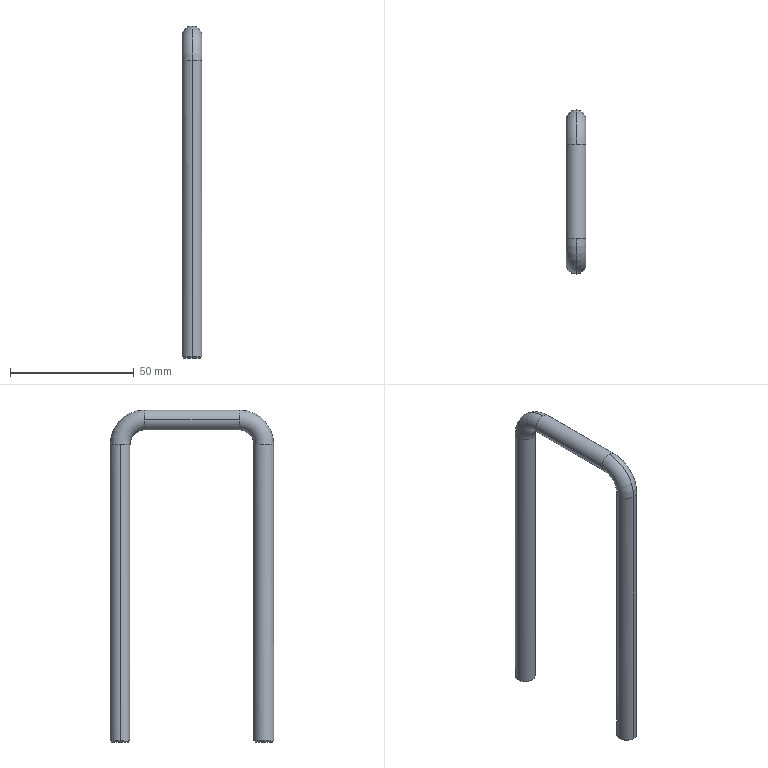Component | SolidWorks | 8x50U-Bolt-1 | 1 solid | 16 faces | box 8 x 66 x 134 mm | volume 15547 mm3 | cylinder 6 | torus 4 | cone 4 | plane 2 | commonest cylinder face diameters 8 x6
build123d program:
from build123d import *

# Parameters (mm, degrees)
SKETCH2_R     = 4
CHAMFER1_SIZE = 0.5


with BuildPart() as part:
    # Sweep1: sweep along a path in Sketch1
    with BuildLine(Plane.XY) as sweep1_path:
        Line((-29, 0), (-29, 120))
        ThreePointArc((-29, 120), (-26.071, 127.071), (-19, 130))
        Line((-19, 130), (19, 130))
        ThreePointArc((19, 130), (26.071, 127.071), (29, 120))
        Line((29, 120), (29, 0))
    # Sketch2 → Sweep1 (sweep)
    with BuildSketch(Plane(origin=(0, 0, 0), x_dir=(1, 0, 0), z_dir=(0, 1, 0))):
        with Locations((-29, 0)):
            Circle(SKETCH2_R)
    sweep(path=sweep1_path.line)

    # Chamfer1
    chamfer1_edges = [part.edges().sort_by_distance(p)[0] for p in [
        (-33, 0, 0),
        (33, 0, 0),
    ]]
    chamfer(chamfer1_edges, length=CHAMFER1_SIZE)


solid = part.part

# Placed as in the assembly
solid = solid.moved(Location((0, -15, -66), (90, -90, 0)))
STEP:
#1=CARTESIAN_POINT('',(-0.,-1.575,2.126));
#2=VERTEX_POINT('',#1);
#3=CARTESIAN_POINT('',(-0.,-1.89,2.126));
#4=VERTEX_POINT('',#3);
#5=CARTESIAN_POINT('',(-0.,-1.732,2.126));
#6=DIRECTION('',(-0.,-0.,1.));
#7=DIRECTION('',(1.,0.,0.));
#8=AXIS2_PLACEMENT_3D('',#5,#6,#7);
#9=CIRCLE('',#8,0.1575);
#10=EDGE_CURVE('',#2,#4,#9,.T.);
#11=ORIENTED_EDGE('',*,*,#10,.T.);
#12=CARTESIAN_POINT('',(-0.,-1.339,2.677));
#13=VERTEX_POINT('',#12);
#14=CARTESIAN_POINT('',(-0.,-1.339,2.126));
#15=DIRECTION('',(-1.,0.,-0.));
#16=DIRECTION('',(-0.,-1.,0.));
#17=AXIS2_PLACEMENT_3D('',#14,#15,#16);
#18=CIRCLE('',#17,0.5512);
#19=EDGE_CURVE('',#4,#13,#18,.T.);
#20=ORIENTED_EDGE('',*,*,#19,.T.);
#21=CARTESIAN_POINT('',(-0.1575,-1.339,2.52));
#22=VERTEX_POINT('',#21);
#23=CARTESIAN_POINT('',(-0.,-1.339,2.52));
#24=DIRECTION('',(0.,1.,0.));
#25=DIRECTION('',(1.,0.,0.));
#26=AXIS2_PLACEMENT_3D('',#23,#24,#25);
#27=CIRCLE('',#26,0.1575);
#28=EDGE_CURVE('',#22,#13,#27,.T.);
#29=ORIENTED_EDGE('',*,*,#28,.F.);
#30=CARTESIAN_POINT('',(-0.,-1.339,2.362));
#31=VERTEX_POINT('',#30);
#32=CARTESIAN_POINT('',(-0.,-1.339,2.52));
#33=DIRECTION('',(0.,1.,0.));
#34=DIRECTION('',(1.,0.,0.));
#35=AXIS2_PLACEMENT_3D('',#32,#33,#34);
#36=CIRCLE('',#35,0.1575);
#37=EDGE_CURVE('',#31,#22,#36,.T.);
#38=ORIENTED_EDGE('',*,*,#37,.F.);
#39=CARTESIAN_POINT('',(-0.,-1.339,2.126));
#40=DIRECTION('',(-1.,0.,-0.));
#41=DIRECTION('',(-0.,-1.,0.));
#42=AXIS2_PLACEMENT_3D('',#39,#40,#41);
#43=CIRCLE('',#42,0.2362);
#44=EDGE_CURVE('',#2,#31,#43,.T.);
#45=ORIENTED_EDGE('',*,*,#44,.F.);
#46=EDGE_LOOP('',(#11,#20,#29,#38,#45));
#47=FACE_OUTER_BOUND('',#46,.T.);
#48=CARTESIAN_POINT('',(-0.,-1.339,2.126));
#49=DIRECTION('',(-1.,0.,-0.));
#50=DIRECTION('',(-0.,-1.,-0.));
#51=AXIS2_PLACEMENT_3D('',#48,#49,#50);
#52=TOROIDAL_SURFACE('',#51,0.3937,0.1575);
#53=ADVANCED_FACE('',(#47),#52,.T.);
#54=CARTESIAN_POINT('',(-0.1575,0.1575,2.52));
#55=VERTEX_POINT('',#54);
#56=CARTESIAN_POINT('',(-0.,0.1575,2.677));
#57=VERTEX_POINT('',#56);
#58=CARTESIAN_POINT('',(-0.,0.1575,2.52));
#59=DIRECTION('',(0.,1.,0.));
#60=DIRECTION('',(1.,0.,0.));
#61=AXIS2_PLACEMENT_3D('',#58,#59,#60);
#62=CIRCLE('',#61,0.1575);
#63=EDGE_CURVE('',#55,#57,#62,.T.);
#64=ORIENTED_EDGE('',*,*,#63,.T.);
#65=CARTESIAN_POINT('',(-0.,0.7087,2.126));
#66=VERTEX_POINT('',#65);
#67=CARTESIAN_POINT('',(-0.,0.1575,2.126));
#68=DIRECTION('',(-1.,0.,-0.));
#69=DIRECTION('',(-0.,-1.,0.));
#70=AXIS2_PLACEMENT_3D('',#67,#68,#69);
#71=CIRCLE('',#70,0.5512);
#72=EDGE_CURVE('',#57,#66,#71,.T.);
#73=ORIENTED_EDGE('',*,*,#72,.T.);
#74=CARTESIAN_POINT('',(-0.1575,0.5512,2.126));
#75=VERTEX_POINT('',#74);
#76=CARTESIAN_POINT('',(-0.,0.5512,2.126));
#77=DIRECTION('',(0.,0.,-1.));
#78=DIRECTION('',(1.,0.,0.));
#79=AXIS2_PLACEMENT_3D('',#76,#77,#78);
#80=CIRCLE('',#79,0.1575);
#81=EDGE_CURVE('',#75,#66,#80,.T.);
#82=ORIENTED_EDGE('',*,*,#81,.F.);
#83=CARTESIAN_POINT('',(-0.,0.3937,2.126));
#84=VERTEX_POINT('',#83);
#85=CARTESIAN_POINT('',(-0.,0.5512,2.126));
#86=DIRECTION('',(0.,0.,-1.));
#87=DIRECTION('',(1.,0.,0.));
#88=AXIS2_PLACEMENT_3D('',#85,#86,#87);
#89=CIRCLE('',#88,0.1575);
#90=EDGE_CURVE('',#84,#75,#89,.T.);
#91=ORIENTED_EDGE('',*,*,#90,.F.);
#92=CARTESIAN_POINT('',(-0.,0.1575,2.362));
#93=VERTEX_POINT('',#92);
#94=CARTESIAN_POINT('',(-0.,0.1575,2.126));
#95=DIRECTION('',(-1.,0.,-0.));
#96=DIRECTION('',(-0.,-1.,0.));
#97=AXIS2_PLACEMENT_3D('',#94,#95,#96);
#98=CIRCLE('',#97,0.2362);
#99=EDGE_CURVE('',#93,#84,#98,.T.);
#100=ORIENTED_EDGE('',*,*,#99,.F.);
#101=CARTESIAN_POINT('',(-0.,0.1575,2.52));
#102=DIRECTION('',(0.,1.,0.));
#103=DIRECTION('',(1.,0.,0.));
#104=AXIS2_PLACEMENT_3D('',#101,#102,#103);
#105=CIRCLE('',#104,0.1575);
#106=EDGE_CURVE('',#93,#55,#105,.T.);
#107=ORIENTED_EDGE('',*,*,#106,.T.);
#108=EDGE_LOOP('',(#64,#73,#82,#91,#100,#107));
#109=FACE_OUTER_BOUND('',#108,.T.);
#110=CARTESIAN_POINT('',(-0.,0.1575,2.126));
#111=DIRECTION('',(-1.,0.,-0.));
#112=DIRECTION('',(-0.,-1.,-0.));
#113=AXIS2_PLACEMENT_3D('',#110,#111,#112);
#114=TOROIDAL_SURFACE('',#113,0.3937,0.1575);
#115=ADVANCED_FACE('',(#109),#114,.T.);
#116=CARTESIAN_POINT('',(-0.1378,-1.732,-2.598));
#117=VERTEX_POINT('',#116);
#118=CARTESIAN_POINT('',(0.1378,-1.732,-2.598));
#119=VERTEX_POINT('',#118);
#120=CARTESIAN_POINT('',(-0.,-1.732,-2.598));
#121=DIRECTION('',(0.,0.,-1.));
#122=DIRECTION('',(1.,0.,0.));
#123=AXIS2_PLACEMENT_3D('',#120,#121,#122);
#124=CIRCLE('',#123,0.1378);
#125=EDGE_CURVE('',#117,#119,#124,.T.);
#126=ORIENTED_EDGE('',*,*,#125,.F.);
#127=CARTESIAN_POINT('',(-0.1575,-1.732,-2.579));
#128=VERTEX_POINT('',#127);
#129=CARTESIAN_POINT('',(-0.1575,-1.732,-2.579));
#130=DIRECTION('',(-0.7071,0.,0.7071));
#131=VECTOR('',#130,39.37);
#132=LINE('',#129,#131);
#133=EDGE_CURVE('',#117,#128,#132,.T.);
#134=ORIENTED_EDGE('',*,*,#133,.T.);
#135=CARTESIAN_POINT('',(-0.,-1.575,-2.579));
#136=VERTEX_POINT('',#135);
#137=CARTESIAN_POINT('',(-0.,-1.732,-2.579));
#138=DIRECTION('',(-0.,-0.,1.));
#139=DIRECTION('',(1.,0.,0.));
#140=AXIS2_PLACEMENT_3D('',#137,#138,#139);
#141=CIRCLE('',#140,0.1575);
#142=EDGE_CURVE('',#136,#128,#141,.T.);
#143=ORIENTED_EDGE('',*,*,#142,.F.);
#144=CARTESIAN_POINT('',(0.1575,-1.732,-2.579));
#145=VERTEX_POINT('',#144);
#146=CARTESIAN_POINT('',(-0.,-1.732,-2.579));
#147=DIRECTION('',(-0.,-0.,1.));
#148=DIRECTION('',(1.,0.,0.));
#149=AXIS2_PLACEMENT_3D('',#146,#147,#148);
#150=CIRCLE('',#149,0.1575);
#151=EDGE_CURVE('',#145,#136,#150,.T.);
#152=ORIENTED_EDGE('',*,*,#151,.F.);
#153=CARTESIAN_POINT('',(0.1575,-1.732,-2.579));
#154=DIRECTION('',(0.7071,-0.,0.7071));
#155=VECTOR('',#154,39.37);
#156=LINE('',#153,#155);
#157=EDGE_CURVE('',#119,#145,#156,.T.);
#158=ORIENTED_EDGE('',*,*,#157,.F.);
#159=EDGE_LOOP('',(#126,#134,#143,#152,#158));
#160=FACE_OUTER_BOUND('',#159,.T.);
#161=CARTESIAN_POINT('',(-0.,-1.732,-2.579));
#162=DIRECTION('',(-0.,-0.,1.));
#163=DIRECTION('',(1.,0.,0.));
#164=AXIS2_PLACEMENT_3D('',#161,#162,#163);
#165=CONICAL_SURFACE('',#164,0.1575,0.7854);
#166=ADVANCED_FACE('',(#160),#165,.T.);
#167=CARTESIAN_POINT('',(-0.1378,0.5512,-2.598));
#168=VERTEX_POINT('',#167);
#169=CARTESIAN_POINT('',(0.1378,0.5512,-2.598));
#170=VERTEX_POINT('',#169);
#171=CARTESIAN_POINT('',(-0.,0.5512,-2.598));
#172=DIRECTION('',(0.,0.,-1.));
#173=DIRECTION('',(0.,1.,0.));
#174=AXIS2_PLACEMENT_3D('',#171,#172,#173);
#175=CIRCLE('',#174,0.1378);
#176=EDGE_CURVE('',#168,#170,#175,.T.);
#177=ORIENTED_EDGE('',*,*,#176,.F.);
#178=CARTESIAN_POINT('',(-0.1575,0.5512,-2.579));
#179=VERTEX_POINT('',#178);
#180=CARTESIAN_POINT('',(-0.1378,0.5512,-2.598));
#181=DIRECTION('',(-0.7071,0.,0.7071));
#182=VECTOR('',#181,39.37);
#183=LINE('',#180,#182);
#184=EDGE_CURVE('',#168,#179,#183,.T.);
#185=ORIENTED_EDGE('',*,*,#184,.T.);
#186=CARTESIAN_POINT('',(0.1575,0.5512,-2.579));
#187=VERTEX_POINT('',#186);
#188=CARTESIAN_POINT('',(-0.,0.5512,-2.579));
#189=DIRECTION('',(-0.,-0.,1.));
#190=DIRECTION('',(-1.,0.,0.));
#191=AXIS2_PLACEMENT_3D('',#188,#189,#190);
#192=CIRCLE('',#191,0.1575);
#193=EDGE_CURVE('',#187,#179,#192,.T.);
#194=ORIENTED_EDGE('',*,*,#193,.F.);
#195=CARTESIAN_POINT('',(0.1378,0.5512,-2.598));
#196=DIRECTION('',(0.7071,-0.,0.7071));
#197=VECTOR('',#196,39.37);
#198=LINE('',#195,#197);
#199=EDGE_CURVE('',#170,#187,#198,.T.);
#200=ORIENTED_EDGE('',*,*,#199,.F.);
#201=EDGE_LOOP('',(#177,#185,#194,#200));
#202=FACE_OUTER_BOUND('',#201,.T.);
#203=CARTESIAN_POINT('',(-0.,0.5512,-2.598));
#204=DIRECTION('',(-0.,-0.,1.));
#205=DIRECTION('',(1.,0.,0.));
#206=AXIS2_PLACEMENT_3D('',#203,#204,#205);
#207=CONICAL_SURFACE('',#206,0.1378,0.7854);
#208=ADVANCED_FACE('',(#202),#207,.T.);
#209=CARTESIAN_POINT('',(-0.,-1.732,2.126));
#210=DIRECTION('',(-0.,-0.,1.));
#211=DIRECTION('',(1.,0.,0.));
#212=AXIS2_PLACEMENT_3D('',#209,#210,#211);
#213=CIRCLE('',#212,0.1575);
#214=EDGE_CURVE('',#4,#2,#213,.T.);
#215=ORIENTED_EDGE('',*,*,#214,.F.);
#216=CARTESIAN_POINT('',(-0.,-1.89,-2.579));
#217=VERTEX_POINT('',#216);
#218=CARTESIAN_POINT('',(-0.,-1.89,2.126));
#219=DIRECTION('',(0.,0.,-1.));
#220=VECTOR('',#219,39.37);
#221=LINE('',#218,#220);
#222=EDGE_CURVE('',#4,#217,#221,.T.);
#223=ORIENTED_EDGE('',*,*,#222,.T.);
#224=CARTESIAN_POINT('',(-0.,-1.732,-2.579));
#225=DIRECTION('',(-0.,-0.,1.));
#226=DIRECTION('',(1.,0.,0.));
#227=AXIS2_PLACEMENT_3D('',#224,#225,#226);
#228=CIRCLE('',#227,0.1575);
#229=EDGE_CURVE('',#217,#145,#228,.T.);
#230=ORIENTED_EDGE('',*,*,#229,.T.);
#231=ORIENTED_EDGE('',*,*,#151,.T.);
#232=CARTESIAN_POINT('',(-0.,-1.575,2.126));
#233=DIRECTION('',(0.,0.,-1.));
#234=VECTOR('',#233,39.37);
#235=LINE('',#232,#234);
#236=EDGE_CURVE('',#2,#136,#235,.T.);
#237=ORIENTED_EDGE('',*,*,#236,.F.);
#238=EDGE_LOOP('',(#215,#223,#230,#231,#237));
#239=FACE_OUTER_BOUND('',#238,.T.);
#240=CARTESIAN_POINT('',(-0.,-1.732,2.126));
#241=DIRECTION('',(0.,0.,-1.));
#242=DIRECTION('',(0.,1.,0.));
#243=AXIS2_PLACEMENT_3D('',#240,#241,#242);
#244=CYLINDRICAL_SURFACE('',#243,0.1575);
#245=ADVANCED_FACE('',(#239),#244,.T.);
#246=ORIENTED_EDGE('',*,*,#28,.T.);
#247=CARTESIAN_POINT('',(0.1575,-1.339,2.52));
#248=VERTEX_POINT('',#247);
#249=CARTESIAN_POINT('',(-0.,-1.339,2.52));
#250=DIRECTION('',(0.,1.,0.));
#251=DIRECTION('',(1.,0.,0.));
#252=AXIS2_PLACEMENT_3D('',#249,#250,#251);
#253=CIRCLE('',#252,0.1575);
#254=EDGE_CURVE('',#13,#248,#253,.T.);
#255=ORIENTED_EDGE('',*,*,#254,.T.);
#256=CARTESIAN_POINT('',(0.1575,0.1575,2.52));
#257=VERTEX_POINT('',#256);
#258=CARTESIAN_POINT('',(0.1575,-1.339,2.52));
#259=DIRECTION('',(0.,1.,0.));
#260=VECTOR('',#259,39.37);
#261=LINE('',#258,#260);
#262=EDGE_CURVE('',#248,#257,#261,.T.);
#263=ORIENTED_EDGE('',*,*,#262,.T.);
#264=CARTESIAN_POINT('',(-0.,0.1575,2.52));
#265=DIRECTION('',(0.,1.,0.));
#266=DIRECTION('',(1.,0.,0.));
#267=AXIS2_PLACEMENT_3D('',#264,#265,#266);
#268=CIRCLE('',#267,0.1575);
#269=EDGE_CURVE('',#57,#257,#268,.T.);
#270=ORIENTED_EDGE('',*,*,#269,.F.);
#271=ORIENTED_EDGE('',*,*,#63,.F.);
#272=CARTESIAN_POINT('',(-0.1575,-1.339,2.52));
#273=DIRECTION('',(0.,1.,0.));
#274=VECTOR('',#273,39.37);
#275=LINE('',#272,#274);
#276=EDGE_CURVE('',#22,#55,#275,.T.);
#277=ORIENTED_EDGE('',*,*,#276,.F.);
#278=EDGE_LOOP('',(#246,#255,#263,#270,#271,#277));
#279=FACE_OUTER_BOUND('',#278,.T.);
#280=CARTESIAN_POINT('',(-0.,-1.339,2.52));
#281=DIRECTION('',(0.,1.,0.));
#282=DIRECTION('',(-1.,0.,0.));
#283=AXIS2_PLACEMENT_3D('',#280,#281,#282);
#284=CYLINDRICAL_SURFACE('',#283,0.1575);
#285=ADVANCED_FACE('',(#279),#284,.T.);
#286=ORIENTED_EDGE('',*,*,#81,.T.);
#287=CARTESIAN_POINT('',(0.1575,0.5512,2.126));
#288=VERTEX_POINT('',#287);
#289=CARTESIAN_POINT('',(-0.,0.5512,2.126));
#290=DIRECTION('',(0.,0.,-1.));
#291=DIRECTION('',(1.,0.,0.));
#292=AXIS2_PLACEMENT_3D('',#289,#290,#291);
#293=CIRCLE('',#292,0.1575);
#294=EDGE_CURVE('',#66,#288,#293,.T.);
#295=ORIENTED_EDGE('',*,*,#294,.T.);
#296=CARTESIAN_POINT('',(0.1575,0.5512,2.126));
#297=DIRECTION('',(0.,0.,-1.));
#298=VECTOR('',#297,39.37);
#299=LINE('',#296,#298);
#300=EDGE_CURVE('',#288,#187,#299,.T.);
#301=ORIENTED_EDGE('',*,*,#300,.T.);
#302=ORIENTED_EDGE('',*,*,#193,.T.);
#303=CARTESIAN_POINT('',(-0.1575,0.5512,2.126));
#304=DIRECTION('',(0.,0.,-1.));
#305=VECTOR('',#304,39.37);
#306=LINE('',#303,#305);
#307=EDGE_CURVE('',#75,#179,#306,.T.);
#308=ORIENTED_EDGE('',*,*,#307,.F.);
#309=EDGE_LOOP('',(#286,#295,#301,#302,#308));
#310=FACE_OUTER_BOUND('',#309,.T.);
#311=CARTESIAN_POINT('',(-0.,0.5512,2.126));
#312=DIRECTION('',(0.,0.,-1.));
#313=DIRECTION('',(-1.,0.,0.));
#314=AXIS2_PLACEMENT_3D('',#311,#312,#313);
#315=CYLINDRICAL_SURFACE('',#314,0.1575);
#316=ADVANCED_FACE('',(#310),#315,.T.);
#317=ORIENTED_EDGE('',*,*,#300,.F.);
#318=CARTESIAN_POINT('',(-0.,0.5512,2.126));
#319=DIRECTION('',(0.,0.,-1.));
#320=DIRECTION('',(1.,0.,0.));
#321=AXIS2_PLACEMENT_3D('',#318,#319,#320);
#322=CIRCLE('',#321,0.1575);
#323=EDGE_CURVE('',#288,#84,#322,.T.);
#324=ORIENTED_EDGE('',*,*,#323,.T.);
#325=ORIENTED_EDGE('',*,*,#90,.T.);
#326=ORIENTED_EDGE('',*,*,#307,.T.);
#327=CARTESIAN_POINT('',(-0.,0.5512,-2.579));
#328=DIRECTION('',(-0.,-0.,1.));
#329=DIRECTION('',(-1.,0.,0.));
#330=AXIS2_PLACEMENT_3D('',#327,#328,#329);
#331=CIRCLE('',#330,0.1575);
#332=EDGE_CURVE('',#179,#187,#331,.T.);
#333=ORIENTED_EDGE('',*,*,#332,.T.);
#334=EDGE_LOOP('',(#317,#324,#325,#326,#333));
#335=FACE_OUTER_BOUND('',#334,.T.);
#336=CARTESIAN_POINT('',(-0.,0.5512,2.126));
#337=DIRECTION('',(0.,0.,-1.));
#338=DIRECTION('',(-1.,0.,0.));
#339=AXIS2_PLACEMENT_3D('',#336,#337,#338);
#340=CYLINDRICAL_SURFACE('',#339,0.1575);
#341=ADVANCED_FACE('',(#335),#340,.T.);
#342=ORIENTED_EDGE('',*,*,#72,.F.);
#343=ORIENTED_EDGE('',*,*,#269,.T.);
#344=CARTESIAN_POINT('',(-0.,0.1575,2.52));
#345=DIRECTION('',(0.,1.,0.));
#346=DIRECTION('',(1.,0.,0.));
#347=AXIS2_PLACEMENT_3D('',#344,#345,#346);
#348=CIRCLE('',#347,0.1575);
#349=EDGE_CURVE('',#257,#93,#348,.T.);
#350=ORIENTED_EDGE('',*,*,#349,.T.);
#351=ORIENTED_EDGE('',*,*,#99,.T.);
#352=ORIENTED_EDGE('',*,*,#323,.F.);
#353=ORIENTED_EDGE('',*,*,#294,.F.);
#354=EDGE_LOOP('',(#342,#343,#350,#351,#352,#353));
#355=FACE_OUTER_BOUND('',#354,.T.);
#356=CARTESIAN_POINT('',(-0.,0.1575,2.126));
#357=DIRECTION('',(-1.,0.,-0.));
#358=DIRECTION('',(-0.,-1.,-0.));
#359=AXIS2_PLACEMENT_3D('',#356,#357,#358);
#360=TOROIDAL_SURFACE('',#359,0.3937,0.1575);
#361=ADVANCED_FACE('',(#355),#360,.T.);
#362=ORIENTED_EDGE('',*,*,#262,.F.);
#363=CARTESIAN_POINT('',(-0.,-1.339,2.52));
#364=DIRECTION('',(0.,1.,0.));
#365=DIRECTION('',(1.,0.,0.));
#366=AXIS2_PLACEMENT_3D('',#363,#364,#365);
#367=CIRCLE('',#366,0.1575);
#368=EDGE_CURVE('',#248,#31,#367,.T.);
#369=ORIENTED_EDGE('',*,*,#368,.T.);
#370=ORIENTED_EDGE('',*,*,#37,.T.);
#371=ORIENTED_EDGE('',*,*,#276,.T.);
#372=ORIENTED_EDGE('',*,*,#106,.F.);
#373=ORIENTED_EDGE('',*,*,#349,.F.);
#374=EDGE_LOOP('',(#362,#369,#370,#371,#372,#373));
#375=FACE_OUTER_BOUND('',#374,.T.);
#376=CARTESIAN_POINT('',(-0.,-1.339,2.52));
#377=DIRECTION('',(0.,1.,0.));
#378=DIRECTION('',(-1.,0.,0.));
#379=AXIS2_PLACEMENT_3D('',#376,#377,#378);
#380=CYLINDRICAL_SURFACE('',#379,0.1575);
#381=ADVANCED_FACE('',(#375),#380,.T.);
#382=ORIENTED_EDGE('',*,*,#19,.F.);
#383=ORIENTED_EDGE('',*,*,#214,.T.);
#384=ORIENTED_EDGE('',*,*,#44,.T.);
#385=ORIENTED_EDGE('',*,*,#368,.F.);
#386=ORIENTED_EDGE('',*,*,#254,.F.);
#387=EDGE_LOOP('',(#382,#383,#384,#385,#386));
#388=FACE_OUTER_BOUND('',#387,.T.);
#389=CARTESIAN_POINT('',(-0.,-1.339,2.126));
#390=DIRECTION('',(-1.,0.,-0.));
#391=DIRECTION('',(-0.,-1.,-0.));
#392=AXIS2_PLACEMENT_3D('',#389,#390,#391);
#393=TOROIDAL_SURFACE('',#392,0.3937,0.1575);
#394=ADVANCED_FACE('',(#388),#393,.T.);
#395=ORIENTED_EDGE('',*,*,#222,.F.);
#396=ORIENTED_EDGE('',*,*,#10,.F.);
#397=ORIENTED_EDGE('',*,*,#236,.T.);
#398=ORIENTED_EDGE('',*,*,#142,.T.);
#399=CARTESIAN_POINT('',(-0.,-1.732,-2.579));
#400=DIRECTION('',(-0.,-0.,1.));
#401=DIRECTION('',(1.,0.,0.));
#402=AXIS2_PLACEMENT_3D('',#399,#400,#401);
#403=CIRCLE('',#402,0.1575);
#404=EDGE_CURVE('',#128,#217,#403,.T.);
#405=ORIENTED_EDGE('',*,*,#404,.T.);
#406=EDGE_LOOP('',(#395,#396,#397,#398,#405));
#407=FACE_OUTER_BOUND('',#406,.T.);
#408=CARTESIAN_POINT('',(-0.,-1.732,2.126));
#409=DIRECTION('',(0.,0.,-1.));
#410=DIRECTION('',(0.,1.,0.));
#411=AXIS2_PLACEMENT_3D('',#408,#409,#410);
#412=CYLINDRICAL_SURFACE('',#411,0.1575);
#413=ADVANCED_FACE('',(#407),#412,.T.);
#414=CARTESIAN_POINT('',(-0.,0.5512,-2.598));
#415=DIRECTION('',(0.,0.,-1.));
#416=DIRECTION('',(0.,1.,0.));
#417=AXIS2_PLACEMENT_3D('',#414,#415,#416);
#418=CIRCLE('',#417,0.1378);
#419=EDGE_CURVE('',#170,#168,#418,.T.);
#420=ORIENTED_EDGE('',*,*,#419,.T.);
#421=ORIENTED_EDGE('',*,*,#176,.T.);
#422=EDGE_LOOP('',(#420,#421));
#423=FACE_OUTER_BOUND('',#422,.T.);
#424=CARTESIAN_POINT('',(-0.,0.5512,-2.598));
#425=DIRECTION('',(0.,0.,-1.));
#426=DIRECTION('',(1.,-0.,0.));
#427=AXIS2_PLACEMENT_3D('',#424,#425,#426);
#428=PLANE('',#427);
#429=ADVANCED_FACE('',(#423),#428,.T.);
#430=CARTESIAN_POINT('',(-0.,-1.732,-2.598));
#431=DIRECTION('',(0.,0.,-1.));
#432=DIRECTION('',(1.,0.,0.));
#433=AXIS2_PLACEMENT_3D('',#430,#431,#432);
#434=CIRCLE('',#433,0.1378);
#435=EDGE_CURVE('',#119,#117,#434,.T.);
#436=ORIENTED_EDGE('',*,*,#435,.T.);
#437=ORIENTED_EDGE('',*,*,#125,.T.);
#438=EDGE_LOOP('',(#436,#437));
#439=FACE_OUTER_BOUND('',#438,.T.);
#440=CARTESIAN_POINT('',(-0.,-1.732,-2.598));
#441=DIRECTION('',(-0.,-0.,1.));
#442=DIRECTION('',(1.,-0.,0.));
#443=AXIS2_PLACEMENT_3D('',#440,#441,#442);
#444=PLANE('',#443);
#445=ADVANCED_FACE('',(#439),#444,.F.);
#446=ORIENTED_EDGE('',*,*,#184,.F.);
#447=ORIENTED_EDGE('',*,*,#419,.F.);
#448=ORIENTED_EDGE('',*,*,#199,.T.);
#449=ORIENTED_EDGE('',*,*,#332,.F.);
#450=EDGE_LOOP('',(#446,#447,#448,#449));
#451=FACE_OUTER_BOUND('',#450,.T.);
#452=CARTESIAN_POINT('',(-0.,0.5512,-2.598));
#453=DIRECTION('',(-0.,-0.,1.));
#454=DIRECTION('',(1.,0.,0.));
#455=AXIS2_PLACEMENT_3D('',#452,#453,#454);
#456=CONICAL_SURFACE('',#455,0.1378,0.7854);
#457=ADVANCED_FACE('',(#451),#456,.T.);
#458=ORIENTED_EDGE('',*,*,#133,.F.);
#459=ORIENTED_EDGE('',*,*,#435,.F.);
#460=ORIENTED_EDGE('',*,*,#157,.T.);
#461=ORIENTED_EDGE('',*,*,#229,.F.);
#462=ORIENTED_EDGE('',*,*,#404,.F.);
#463=EDGE_LOOP('',(#458,#459,#460,#461,#462));
#464=FACE_OUTER_BOUND('',#463,.T.);
#465=CARTESIAN_POINT('',(-0.,-1.732,-2.579));
#466=DIRECTION('',(-0.,-0.,1.));
#467=DIRECTION('',(1.,0.,0.));
#468=AXIS2_PLACEMENT_3D('',#465,#466,#467);
#469=CONICAL_SURFACE('',#468,0.1575,0.7854);
#470=ADVANCED_FACE('',(#464),#469,.T.);
#471=CLOSED_SHELL('',(#53,#115,#166,#208,#245,#285,#316,#341,#361,#381,#394,#413,#429,#445,#457,#470));
#472=MANIFOLD_SOLID_BREP('',#471);
#473=CARTESIAN_POINT('',(0.,0.,0.));
#474=DIRECTION('',(0.,0.,1.));
#475=DIRECTION('',(1.,0.,0.));
#476=AXIS2_PLACEMENT_3D('',#473,#474,#475);
#477=(LENGTH_UNIT()NAMED_UNIT(*)SI_UNIT($,.METRE.));
#478=LENGTH_MEASURE_WITH_UNIT(LENGTH_MEASURE(0.0254),#477);
#479=DIMENSIONAL_EXPONENTS(1.,0.,0.,0.,0.,0.,0.);
#480=(CONVERSION_BASED_UNIT('',#478)LENGTH_UNIT()NAMED_UNIT(#479));
#481=UNCERTAINTY_MEASURE_WITH_UNIT(LENGTH_MEASURE(0.00001),#480,'','');
#482=(NAMED_UNIT(*)PLANE_ANGLE_UNIT()SI_UNIT($,.RADIAN.));
#483=(NAMED_UNIT(*)SI_UNIT($,.STERADIAN.)SOLID_ANGLE_UNIT());
#484=(GEOMETRIC_REPRESENTATION_CONTEXT(3)GLOBAL_UNCERTAINTY_ASSIGNED_CONTEXT((#481))GLOBAL_UNIT_ASSIGNED_CONTEXT((#480,#482,#483))REPRESENTATION_CONTEXT('',''));
#485=ADVANCED_BREP_SHAPE_REPRESENTATION('',(#472,#476),#484);
#486=COLOUR_RGB('',0.7922,0.8196,0.9333);
#487=FILL_AREA_STYLE_COLOUR('',#486);
#488=FILL_AREA_STYLE('',(#487));
#489=SURFACE_STYLE_FILL_AREA(#488);
#490=SURFACE_SIDE_STYLE('',(#489));
#491=SURFACE_STYLE_USAGE(.BOTH.,#490);
#492=PRESENTATION_STYLE_ASSIGNMENT((#491));
#493=STYLED_ITEM('',(#492),#472);
#494=(LENGTH_UNIT()NAMED_UNIT(*)SI_UNIT($,.METRE.));
#495=LENGTH_MEASURE_WITH_UNIT(LENGTH_MEASURE(0.0254),#494);
#496=DIMENSIONAL_EXPONENTS(1.,0.,0.,0.,0.,0.,0.);
#497=(CONVERSION_BASED_UNIT('',#495)LENGTH_UNIT()NAMED_UNIT(#496));
#498=UNCERTAINTY_MEASURE_WITH_UNIT(LENGTH_MEASURE(0.00001),#497,'','');
#499=(NAMED_UNIT(*)PLANE_ANGLE_UNIT()SI_UNIT($,.RADIAN.));
#500=(NAMED_UNIT(*)SI_UNIT($,.STERADIAN.)SOLID_ANGLE_UNIT());
#501=(GEOMETRIC_REPRESENTATION_CONTEXT(3)GLOBAL_UNCERTAINTY_ASSIGNED_CONTEXT((#498))GLOBAL_UNIT_ASSIGNED_CONTEXT((#497,#499,#500))REPRESENTATION_CONTEXT('',''));
#502=MECHANICAL_DESIGN_GEOMETRIC_PRESENTATION_REPRESENTATION('',(#493),#501);
#503=PRESENTATION_LAYER_ASSIGNMENT('','',(#493));